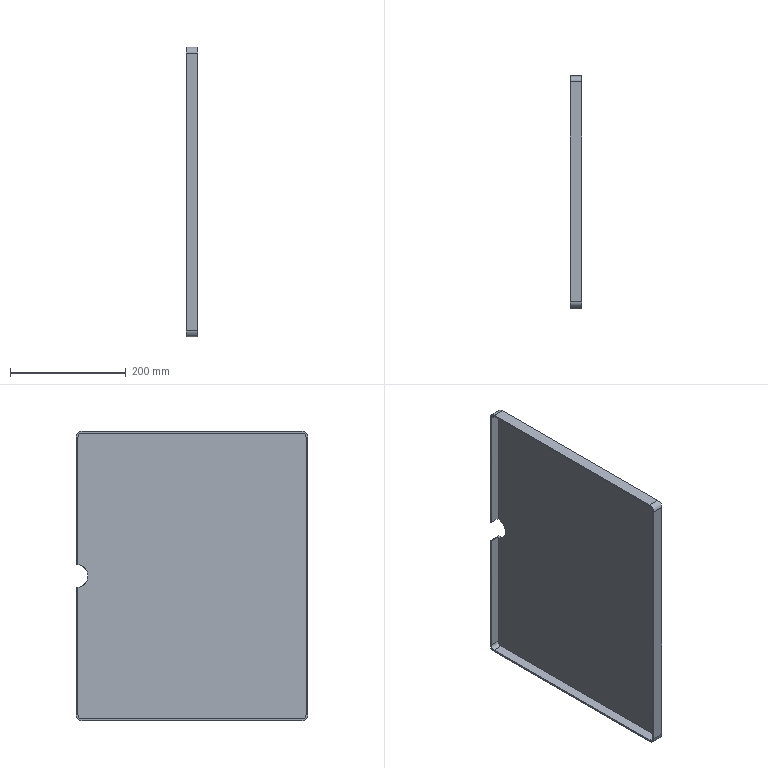Component | SolidWorks | LX-TSJ-17-1 | 1 solid | 22 faces | box 20 x 400 x 500 mm | volume 686219 mm3 | plane 13 | cylinder 9 | commonest cylinder face diameters 20 x4 14 x4 40.343 x1
STEP:
#1=COLOUR_RGB('',0.7922,0.8196,0.9333);
#2=FILL_AREA_STYLE_COLOUR('',#1);
#3=FILL_AREA_STYLE('',(#2));
#4=SURFACE_STYLE_FILL_AREA(#3);
#5=SURFACE_SIDE_STYLE('',(#4));
#6=SURFACE_STYLE_USAGE(.BOTH.,#5);
#7=PRESENTATION_STYLE_ASSIGNMENT((#6));
#8=CARTESIAN_POINT('',(4.999,-15.234,-15.481));
#9=VERTEX_POINT('',#8);
#10=CARTESIAN_POINT('',(4.999,-15.234,-17.069));
#11=VERTEX_POINT('',#10);
#12=CARTESIAN_POINT('',(4.999,-15.234,-16.275));
#13=DIRECTION('',(1.,0.,-0.));
#14=DIRECTION('',(-0.,0.,-1.));
#15=AXIS2_PLACEMENT_3D('',#12,#13,#14);
#16=CIRCLE('',#15,0.7941);
#17=EDGE_CURVE('',#9,#11,#16,.T.);
#18=ORIENTED_EDGE('',*,*,#17,.F.);
#19=CARTESIAN_POINT('',(4.999,-15.234,-6.826));
#20=VERTEX_POINT('',#19);
#21=CARTESIAN_POINT('',(4.999,-15.234,-25.724));
#22=DIRECTION('',(-0.,0.,-1.));
#23=VECTOR('',#22,39.37);
#24=LINE('',#21,#23);
#25=EDGE_CURVE('',#20,#9,#24,.T.);
#26=ORIENTED_EDGE('',*,*,#25,.F.);
#27=CARTESIAN_POINT('',(4.999,-15.627,-6.433));
#28=VERTEX_POINT('',#27);
#29=CARTESIAN_POINT('',(4.999,-15.627,-6.826));
#30=DIRECTION('',(-1.,0.,0.));
#31=DIRECTION('',(-0.,0.,-1.));
#32=AXIS2_PLACEMENT_3D('',#29,#30,#31);
#33=CIRCLE('',#32,0.3937);
#34=EDGE_CURVE('',#28,#20,#33,.T.);
#35=ORIENTED_EDGE('',*,*,#34,.F.);
#36=CARTESIAN_POINT('',(4.999,-30.588,-6.433));
#37=VERTEX_POINT('',#36);
#38=CARTESIAN_POINT('',(4.999,-30.588,-6.433));
#39=DIRECTION('',(0.,1.,0.));
#40=VECTOR('',#39,39.37);
#41=LINE('',#38,#40);
#42=EDGE_CURVE('',#37,#28,#41,.T.);
#43=ORIENTED_EDGE('',*,*,#42,.F.);
#44=CARTESIAN_POINT('',(4.999,-30.982,-6.826));
#45=VERTEX_POINT('',#44);
#46=CARTESIAN_POINT('',(4.999,-30.588,-6.826));
#47=DIRECTION('',(-1.,0.,0.));
#48=DIRECTION('',(-0.,0.,-1.));
#49=AXIS2_PLACEMENT_3D('',#46,#47,#48);
#50=CIRCLE('',#49,0.3937);
#51=EDGE_CURVE('',#45,#37,#50,.T.);
#52=ORIENTED_EDGE('',*,*,#51,.F.);
#53=CARTESIAN_POINT('',(4.999,-30.982,-25.724));
#54=VERTEX_POINT('',#53);
#55=CARTESIAN_POINT('',(4.999,-30.982,-25.724));
#56=DIRECTION('',(0.,0.,1.));
#57=VECTOR('',#56,39.37);
#58=LINE('',#55,#57);
#59=EDGE_CURVE('',#54,#45,#58,.T.);
#60=ORIENTED_EDGE('',*,*,#59,.F.);
#61=CARTESIAN_POINT('',(4.999,-30.588,-26.118));
#62=VERTEX_POINT('',#61);
#63=CARTESIAN_POINT('',(4.999,-30.588,-25.724));
#64=DIRECTION('',(-1.,0.,0.));
#65=DIRECTION('',(-0.,0.,-1.));
#66=AXIS2_PLACEMENT_3D('',#63,#64,#65);
#67=CIRCLE('',#66,0.3937);
#68=EDGE_CURVE('',#62,#54,#67,.T.);
#69=ORIENTED_EDGE('',*,*,#68,.F.);
#70=CARTESIAN_POINT('',(4.999,-15.627,-26.118));
#71=VERTEX_POINT('',#70);
#72=CARTESIAN_POINT('',(4.999,-30.588,-26.118));
#73=DIRECTION('',(0.,-1.,0.));
#74=VECTOR('',#73,39.37);
#75=LINE('',#72,#74);
#76=EDGE_CURVE('',#71,#62,#75,.T.);
#77=ORIENTED_EDGE('',*,*,#76,.F.);
#78=CARTESIAN_POINT('',(4.999,-15.234,-25.724));
#79=VERTEX_POINT('',#78);
#80=CARTESIAN_POINT('',(4.999,-15.627,-25.724));
#81=DIRECTION('',(-1.,0.,0.));
#82=DIRECTION('',(-0.,0.,-1.));
#83=AXIS2_PLACEMENT_3D('',#80,#81,#82);
#84=CIRCLE('',#83,0.3937);
#85=EDGE_CURVE('',#79,#71,#84,.T.);
#86=ORIENTED_EDGE('',*,*,#85,.F.);
#87=CARTESIAN_POINT('',(4.999,-15.234,-25.724));
#88=DIRECTION('',(-0.,0.,-1.));
#89=VECTOR('',#88,39.37);
#90=LINE('',#87,#89);
#91=EDGE_CURVE('',#11,#79,#90,.T.);
#92=ORIENTED_EDGE('',*,*,#91,.F.);
#93=EDGE_LOOP('',(#18,#26,#35,#43,#52,#60,#69,#77,#86,#92));
#94=FACE_OUTER_BOUND('',#93,.T.);
#95=CARTESIAN_POINT('',(4.999,-30.588,-25.724));
#96=DIRECTION('',(-1.,0.,0.));
#97=DIRECTION('',(0.,0.,1.));
#98=AXIS2_PLACEMENT_3D('',#95,#96,#97);
#99=PLANE('',#98);
#100=ADVANCED_FACE('',(#94),#99,.F.);
#101=CARTESIAN_POINT('',(4.212,-15.234,-17.069));
#102=VERTEX_POINT('',#101);
#103=CARTESIAN_POINT('',(4.212,-15.234,-17.069));
#104=DIRECTION('',(-1.,0.,0.));
#105=VECTOR('',#104,39.37);
#106=LINE('',#103,#105);
#107=EDGE_CURVE('',#11,#102,#106,.T.);
#108=ORIENTED_EDGE('',*,*,#107,.F.);
#109=ORIENTED_EDGE('',*,*,#91,.T.);
#110=CARTESIAN_POINT('',(4.212,-15.234,-25.724));
#111=VERTEX_POINT('',#110);
#112=CARTESIAN_POINT('',(4.212,-15.234,-25.724));
#113=DIRECTION('',(1.,0.,-0.));
#114=VECTOR('',#113,39.37);
#115=LINE('',#112,#114);
#116=EDGE_CURVE('',#111,#79,#115,.T.);
#117=ORIENTED_EDGE('',*,*,#116,.F.);
#118=CARTESIAN_POINT('',(4.212,-15.234,-25.724));
#119=DIRECTION('',(-0.,0.,-1.));
#120=VECTOR('',#119,39.37);
#121=LINE('',#118,#120);
#122=EDGE_CURVE('',#102,#111,#121,.T.);
#123=ORIENTED_EDGE('',*,*,#122,.F.);
#124=EDGE_LOOP('',(#108,#109,#117,#123));
#125=FACE_OUTER_BOUND('',#124,.T.);
#126=CARTESIAN_POINT('',(4.212,-15.234,-25.724));
#127=DIRECTION('',(0.,-1.,0.));
#128=DIRECTION('',(1.,0.,-0.));
#129=AXIS2_PLACEMENT_3D('',#126,#127,#128);
#130=PLANE('',#129);
#131=ADVANCED_FACE('',(#125),#130,.F.);
#132=CARTESIAN_POINT('',(4.881,-15.352,-17.061));
#133=VERTEX_POINT('',#132);
#134=CARTESIAN_POINT('',(4.212,-15.352,-17.061));
#135=VERTEX_POINT('',#134);
#136=CARTESIAN_POINT('',(4.212,-15.352,-17.061));
#137=DIRECTION('',(-1.,0.,0.));
#138=VECTOR('',#137,39.37);
#139=LINE('',#136,#138);
#140=EDGE_CURVE('',#133,#135,#139,.T.);
#141=ORIENTED_EDGE('',*,*,#140,.F.);
#142=CARTESIAN_POINT('',(4.881,-15.352,-15.49));
#143=VERTEX_POINT('',#142);
#144=CARTESIAN_POINT('',(4.881,-15.234,-16.275));
#145=DIRECTION('',(1.,0.,-0.));
#146=DIRECTION('',(-0.,0.,-1.));
#147=AXIS2_PLACEMENT_3D('',#144,#145,#146);
#148=CIRCLE('',#147,0.7941);
#149=EDGE_CURVE('',#143,#133,#148,.T.);
#150=ORIENTED_EDGE('',*,*,#149,.F.);
#151=CARTESIAN_POINT('',(4.212,-15.352,-15.49));
#152=VERTEX_POINT('',#151);
#153=CARTESIAN_POINT('',(4.212,-15.352,-15.49));
#154=DIRECTION('',(1.,0.,-0.));
#155=VECTOR('',#154,39.37);
#156=LINE('',#153,#155);
#157=EDGE_CURVE('',#152,#143,#156,.T.);
#158=ORIENTED_EDGE('',*,*,#157,.F.);
#159=CARTESIAN_POINT('',(4.212,-15.234,-15.481));
#160=VERTEX_POINT('',#159);
#161=CARTESIAN_POINT('',(4.212,-15.234,-16.275));
#162=DIRECTION('',(1.,0.,-0.));
#163=DIRECTION('',(-0.,0.,-1.));
#164=AXIS2_PLACEMENT_3D('',#161,#162,#163);
#165=CIRCLE('',#164,0.7941);
#166=EDGE_CURVE('',#160,#152,#165,.T.);
#167=ORIENTED_EDGE('',*,*,#166,.F.);
#168=CARTESIAN_POINT('',(4.212,-15.234,-15.481));
#169=DIRECTION('',(-1.,0.,0.));
#170=VECTOR('',#169,39.37);
#171=LINE('',#168,#170);
#172=EDGE_CURVE('',#9,#160,#171,.T.);
#173=ORIENTED_EDGE('',*,*,#172,.F.);
#174=ORIENTED_EDGE('',*,*,#17,.T.);
#175=ORIENTED_EDGE('',*,*,#107,.T.);
#176=CARTESIAN_POINT('',(4.212,-15.234,-16.275));
#177=DIRECTION('',(1.,0.,-0.));
#178=DIRECTION('',(-0.,0.,-1.));
#179=AXIS2_PLACEMENT_3D('',#176,#177,#178);
#180=CIRCLE('',#179,0.7941);
#181=EDGE_CURVE('',#135,#102,#180,.T.);
#182=ORIENTED_EDGE('',*,*,#181,.F.);
#183=EDGE_LOOP('',(#141,#150,#158,#167,#173,#174,#175,#182));
#184=FACE_OUTER_BOUND('',#183,.T.);
#185=CARTESIAN_POINT('',(4.212,-15.234,-16.275));
#186=DIRECTION('',(1.,0.,-0.));
#187=DIRECTION('',(-0.,0.,-1.));
#188=AXIS2_PLACEMENT_3D('',#185,#186,#187);
#189=CYLINDRICAL_SURFACE('',#188,0.7941);
#190=ADVANCED_FACE('',(#184),#189,.F.);
#191=ORIENTED_EDGE('',*,*,#172,.T.);
#192=CARTESIAN_POINT('',(4.212,-15.234,-6.826));
#193=VERTEX_POINT('',#192);
#194=CARTESIAN_POINT('',(4.212,-15.234,-25.724));
#195=DIRECTION('',(-0.,0.,-1.));
#196=VECTOR('',#195,39.37);
#197=LINE('',#194,#196);
#198=EDGE_CURVE('',#193,#160,#197,.T.);
#199=ORIENTED_EDGE('',*,*,#198,.F.);
#200=CARTESIAN_POINT('',(4.212,-15.234,-6.826));
#201=DIRECTION('',(-1.,0.,0.));
#202=VECTOR('',#201,39.37);
#203=LINE('',#200,#202);
#204=EDGE_CURVE('',#20,#193,#203,.T.);
#205=ORIENTED_EDGE('',*,*,#204,.F.);
#206=ORIENTED_EDGE('',*,*,#25,.T.);
#207=EDGE_LOOP('',(#191,#199,#205,#206));
#208=FACE_OUTER_BOUND('',#207,.T.);
#209=CARTESIAN_POINT('',(4.212,-15.234,-25.724));
#210=DIRECTION('',(0.,-1.,0.));
#211=DIRECTION('',(1.,0.,-0.));
#212=AXIS2_PLACEMENT_3D('',#209,#210,#211);
#213=PLANE('',#212);
#214=ADVANCED_FACE('',(#208),#213,.F.);
#215=CARTESIAN_POINT('',(4.212,-15.627,-6.433));
#216=VERTEX_POINT('',#215);
#217=CARTESIAN_POINT('',(4.212,-15.627,-6.826));
#218=DIRECTION('',(1.,0.,-0.));
#219=DIRECTION('',(-0.,0.,-1.));
#220=AXIS2_PLACEMENT_3D('',#217,#218,#219);
#221=CIRCLE('',#220,0.3937);
#222=EDGE_CURVE('',#193,#216,#221,.T.);
#223=ORIENTED_EDGE('',*,*,#222,.T.);
#224=CARTESIAN_POINT('',(4.212,-15.627,-6.433));
#225=DIRECTION('',(1.,0.,-0.));
#226=VECTOR('',#225,39.37);
#227=LINE('',#224,#226);
#228=EDGE_CURVE('',#216,#28,#227,.T.);
#229=ORIENTED_EDGE('',*,*,#228,.T.);
#230=ORIENTED_EDGE('',*,*,#34,.T.);
#231=ORIENTED_EDGE('',*,*,#204,.T.);
#232=EDGE_LOOP('',(#223,#229,#230,#231));
#233=FACE_OUTER_BOUND('',#232,.T.);
#234=CARTESIAN_POINT('',(4.212,-15.627,-6.826));
#235=DIRECTION('',(1.,0.,-0.));
#236=DIRECTION('',(-0.,0.,-1.));
#237=AXIS2_PLACEMENT_3D('',#234,#235,#236);
#238=CYLINDRICAL_SURFACE('',#237,0.3937);
#239=ADVANCED_FACE('',(#233),#238,.T.);
#240=ORIENTED_EDGE('',*,*,#228,.F.);
#241=CARTESIAN_POINT('',(4.212,-30.588,-6.433));
#242=VERTEX_POINT('',#241);
#243=CARTESIAN_POINT('',(4.212,-15.627,-6.433));
#244=DIRECTION('',(-0.,1.,-0.));
#245=VECTOR('',#244,39.37);
#246=LINE('',#243,#245);
#247=EDGE_CURVE('',#242,#216,#246,.T.);
#248=ORIENTED_EDGE('',*,*,#247,.F.);
#249=CARTESIAN_POINT('',(4.212,-30.588,-6.433));
#250=DIRECTION('',(-1.,0.,0.));
#251=VECTOR('',#250,39.37);
#252=LINE('',#249,#251);
#253=EDGE_CURVE('',#37,#242,#252,.T.);
#254=ORIENTED_EDGE('',*,*,#253,.F.);
#255=ORIENTED_EDGE('',*,*,#42,.T.);
#256=EDGE_LOOP('',(#240,#248,#254,#255));
#257=FACE_OUTER_BOUND('',#256,.T.);
#258=CARTESIAN_POINT('',(4.212,-15.627,-6.433));
#259=DIRECTION('',(-0.,-0.,-1.));
#260=DIRECTION('',(0.,-1.,0.));
#261=AXIS2_PLACEMENT_3D('',#258,#259,#260);
#262=PLANE('',#261);
#263=ADVANCED_FACE('',(#257),#262,.F.);
#264=CARTESIAN_POINT('',(4.212,-30.982,-6.826));
#265=VERTEX_POINT('',#264);
#266=CARTESIAN_POINT('',(4.212,-30.588,-6.826));
#267=DIRECTION('',(1.,0.,-0.));
#268=DIRECTION('',(-0.,0.,-1.));
#269=AXIS2_PLACEMENT_3D('',#266,#267,#268);
#270=CIRCLE('',#269,0.3937);
#271=EDGE_CURVE('',#242,#265,#270,.T.);
#272=ORIENTED_EDGE('',*,*,#271,.T.);
#273=CARTESIAN_POINT('',(4.212,-30.982,-6.826));
#274=DIRECTION('',(1.,0.,-0.));
#275=VECTOR('',#274,39.37);
#276=LINE('',#273,#275);
#277=EDGE_CURVE('',#265,#45,#276,.T.);
#278=ORIENTED_EDGE('',*,*,#277,.T.);
#279=ORIENTED_EDGE('',*,*,#51,.T.);
#280=ORIENTED_EDGE('',*,*,#253,.T.);
#281=EDGE_LOOP('',(#272,#278,#279,#280));
#282=FACE_OUTER_BOUND('',#281,.T.);
#283=CARTESIAN_POINT('',(4.212,-30.588,-6.826));
#284=DIRECTION('',(1.,0.,-0.));
#285=DIRECTION('',(-0.,0.,-1.));
#286=AXIS2_PLACEMENT_3D('',#283,#284,#285);
#287=CYLINDRICAL_SURFACE('',#286,0.3937);
#288=ADVANCED_FACE('',(#282),#287,.T.);
#289=ORIENTED_EDGE('',*,*,#277,.F.);
#290=CARTESIAN_POINT('',(4.212,-30.982,-25.724));
#291=VERTEX_POINT('',#290);
#292=CARTESIAN_POINT('',(4.212,-30.982,-25.724));
#293=DIRECTION('',(0.,0.,1.));
#294=VECTOR('',#293,39.37);
#295=LINE('',#292,#294);
#296=EDGE_CURVE('',#291,#265,#295,.T.);
#297=ORIENTED_EDGE('',*,*,#296,.F.);
#298=CARTESIAN_POINT('',(4.212,-30.982,-25.724));
#299=DIRECTION('',(-1.,0.,0.));
#300=VECTOR('',#299,39.37);
#301=LINE('',#298,#300);
#302=EDGE_CURVE('',#54,#291,#301,.T.);
#303=ORIENTED_EDGE('',*,*,#302,.F.);
#304=ORIENTED_EDGE('',*,*,#59,.T.);
#305=EDGE_LOOP('',(#289,#297,#303,#304));
#306=FACE_OUTER_BOUND('',#305,.T.);
#307=CARTESIAN_POINT('',(4.212,-30.982,-25.724));
#308=DIRECTION('',(0.,1.,0.));
#309=DIRECTION('',(-1.,0.,0.));
#310=AXIS2_PLACEMENT_3D('',#307,#308,#309);
#311=PLANE('',#310);
#312=ADVANCED_FACE('',(#306),#311,.F.);
#313=CARTESIAN_POINT('',(4.212,-30.588,-26.118));
#314=VERTEX_POINT('',#313);
#315=CARTESIAN_POINT('',(4.212,-30.588,-25.724));
#316=DIRECTION('',(1.,0.,-0.));
#317=DIRECTION('',(-0.,0.,-1.));
#318=AXIS2_PLACEMENT_3D('',#315,#316,#317);
#319=CIRCLE('',#318,0.3937);
#320=EDGE_CURVE('',#291,#314,#319,.T.);
#321=ORIENTED_EDGE('',*,*,#320,.T.);
#322=CARTESIAN_POINT('',(4.212,-30.588,-26.118));
#323=DIRECTION('',(1.,0.,-0.));
#324=VECTOR('',#323,39.37);
#325=LINE('',#322,#324);
#326=EDGE_CURVE('',#314,#62,#325,.T.);
#327=ORIENTED_EDGE('',*,*,#326,.T.);
#328=ORIENTED_EDGE('',*,*,#68,.T.);
#329=ORIENTED_EDGE('',*,*,#302,.T.);
#330=EDGE_LOOP('',(#321,#327,#328,#329));
#331=FACE_OUTER_BOUND('',#330,.T.);
#332=CARTESIAN_POINT('',(4.212,-30.588,-25.724));
#333=DIRECTION('',(1.,0.,-0.));
#334=DIRECTION('',(-0.,0.,-1.));
#335=AXIS2_PLACEMENT_3D('',#332,#333,#334);
#336=CYLINDRICAL_SURFACE('',#335,0.3937);
#337=ADVANCED_FACE('',(#331),#336,.T.);
#338=ORIENTED_EDGE('',*,*,#326,.F.);
#339=CARTESIAN_POINT('',(4.212,-15.627,-26.118));
#340=VERTEX_POINT('',#339);
#341=CARTESIAN_POINT('',(4.212,-15.627,-26.118));
#342=DIRECTION('',(0.,-1.,0.));
#343=VECTOR('',#342,39.37);
#344=LINE('',#341,#343);
#345=EDGE_CURVE('',#340,#314,#344,.T.);
#346=ORIENTED_EDGE('',*,*,#345,.F.);
#347=CARTESIAN_POINT('',(4.212,-15.627,-26.118));
#348=DIRECTION('',(-1.,0.,0.));
#349=VECTOR('',#348,39.37);
#350=LINE('',#347,#349);
#351=EDGE_CURVE('',#71,#340,#350,.T.);
#352=ORIENTED_EDGE('',*,*,#351,.F.);
#353=ORIENTED_EDGE('',*,*,#76,.T.);
#354=EDGE_LOOP('',(#338,#346,#352,#353));
#355=FACE_OUTER_BOUND('',#354,.T.);
#356=CARTESIAN_POINT('',(4.212,-15.627,-26.118));
#357=DIRECTION('',(0.,0.,1.));
#358=DIRECTION('',(-0.,1.,-0.));
#359=AXIS2_PLACEMENT_3D('',#356,#357,#358);
#360=PLANE('',#359);
#361=ADVANCED_FACE('',(#355),#360,.F.);
#362=CARTESIAN_POINT('',(4.212,-15.627,-25.724));
#363=DIRECTION('',(1.,0.,-0.));
#364=DIRECTION('',(-0.,0.,-1.));
#365=AXIS2_PLACEMENT_3D('',#362,#363,#364);
#366=CIRCLE('',#365,0.3937);
#367=EDGE_CURVE('',#340,#111,#366,.T.);
#368=ORIENTED_EDGE('',*,*,#367,.T.);
#369=ORIENTED_EDGE('',*,*,#116,.T.);
#370=ORIENTED_EDGE('',*,*,#85,.T.);
#371=ORIENTED_EDGE('',*,*,#351,.T.);
#372=EDGE_LOOP('',(#368,#369,#370,#371));
#373=FACE_OUTER_BOUND('',#372,.T.);
#374=CARTESIAN_POINT('',(4.212,-15.627,-25.724));
#375=DIRECTION('',(1.,0.,-0.));
#376=DIRECTION('',(-0.,0.,-1.));
#377=AXIS2_PLACEMENT_3D('',#374,#375,#376);
#378=CYLINDRICAL_SURFACE('',#377,0.3937);
#379=ADVANCED_FACE('',(#373),#378,.T.);
#380=CARTESIAN_POINT('',(4.212,-15.627,-26.));
#381=VERTEX_POINT('',#380);
#382=CARTESIAN_POINT('',(4.212,-15.352,-25.724));
#383=VERTEX_POINT('',#382);
#384=CARTESIAN_POINT('',(4.212,-15.627,-25.724));
#385=DIRECTION('',(1.,0.,-0.));
#386=DIRECTION('',(-0.,0.,-1.));
#387=AXIS2_PLACEMENT_3D('',#384,#385,#386);
#388=CIRCLE('',#387,0.2756);
#389=EDGE_CURVE('',#381,#383,#388,.T.);
#390=ORIENTED_EDGE('',*,*,#389,.T.);
#391=CARTESIAN_POINT('',(4.212,-15.352,-25.724));
#392=DIRECTION('',(0.,0.,1.));
#393=VECTOR('',#392,39.37);
#394=LINE('',#391,#393);
#395=EDGE_CURVE('',#383,#135,#394,.T.);
#396=ORIENTED_EDGE('',*,*,#395,.T.);
#397=ORIENTED_EDGE('',*,*,#181,.T.);
#398=ORIENTED_EDGE('',*,*,#122,.T.);
#399=ORIENTED_EDGE('',*,*,#367,.F.);
#400=ORIENTED_EDGE('',*,*,#345,.T.);
#401=ORIENTED_EDGE('',*,*,#320,.F.);
#402=ORIENTED_EDGE('',*,*,#296,.T.);
#403=ORIENTED_EDGE('',*,*,#271,.F.);
#404=ORIENTED_EDGE('',*,*,#247,.T.);
#405=ORIENTED_EDGE('',*,*,#222,.F.);
#406=ORIENTED_EDGE('',*,*,#198,.T.);
#407=ORIENTED_EDGE('',*,*,#166,.T.);
#408=CARTESIAN_POINT('',(4.212,-15.352,-6.826));
#409=VERTEX_POINT('',#408);
#410=CARTESIAN_POINT('',(4.212,-15.352,-25.724));
#411=DIRECTION('',(0.,0.,1.));
#412=VECTOR('',#411,39.37);
#413=LINE('',#410,#412);
#414=EDGE_CURVE('',#152,#409,#413,.T.);
#415=ORIENTED_EDGE('',*,*,#414,.T.);
#416=CARTESIAN_POINT('',(4.212,-15.627,-6.551));
#417=VERTEX_POINT('',#416);
#418=CARTESIAN_POINT('',(4.212,-15.627,-6.826));
#419=DIRECTION('',(1.,0.,-0.));
#420=DIRECTION('',(-0.,0.,-1.));
#421=AXIS2_PLACEMENT_3D('',#418,#419,#420);
#422=CIRCLE('',#421,0.2756);
#423=EDGE_CURVE('',#409,#417,#422,.T.);
#424=ORIENTED_EDGE('',*,*,#423,.T.);
#425=CARTESIAN_POINT('',(4.212,-30.588,-6.551));
#426=VERTEX_POINT('',#425);
#427=CARTESIAN_POINT('',(4.212,-30.588,-6.551));
#428=DIRECTION('',(0.,-1.,0.));
#429=VECTOR('',#428,39.37);
#430=LINE('',#427,#429);
#431=EDGE_CURVE('',#417,#426,#430,.T.);
#432=ORIENTED_EDGE('',*,*,#431,.T.);
#433=CARTESIAN_POINT('',(4.212,-30.864,-6.826));
#434=VERTEX_POINT('',#433);
#435=CARTESIAN_POINT('',(4.212,-30.588,-6.826));
#436=DIRECTION('',(1.,0.,-0.));
#437=DIRECTION('',(-0.,0.,-1.));
#438=AXIS2_PLACEMENT_3D('',#435,#436,#437);
#439=CIRCLE('',#438,0.2756);
#440=EDGE_CURVE('',#426,#434,#439,.T.);
#441=ORIENTED_EDGE('',*,*,#440,.T.);
#442=CARTESIAN_POINT('',(4.212,-30.864,-25.724));
#443=VERTEX_POINT('',#442);
#444=CARTESIAN_POINT('',(4.212,-30.864,-25.724));
#445=DIRECTION('',(-0.,0.,-1.));
#446=VECTOR('',#445,39.37);
#447=LINE('',#444,#446);
#448=EDGE_CURVE('',#434,#443,#447,.T.);
#449=ORIENTED_EDGE('',*,*,#448,.T.);
#450=CARTESIAN_POINT('',(4.212,-30.588,-26.));
#451=VERTEX_POINT('',#450);
#452=CARTESIAN_POINT('',(4.212,-30.588,-25.724));
#453=DIRECTION('',(1.,0.,-0.));
#454=DIRECTION('',(-0.,0.,-1.));
#455=AXIS2_PLACEMENT_3D('',#452,#453,#454);
#456=CIRCLE('',#455,0.2756);
#457=EDGE_CURVE('',#443,#451,#456,.T.);
#458=ORIENTED_EDGE('',*,*,#457,.T.);
#459=CARTESIAN_POINT('',(4.212,-30.588,-26.));
#460=DIRECTION('',(0.,1.,0.));
#461=VECTOR('',#460,39.37);
#462=LINE('',#459,#461);
#463=EDGE_CURVE('',#451,#381,#462,.T.);
#464=ORIENTED_EDGE('',*,*,#463,.T.);
#465=EDGE_LOOP('',(#390,#396,#397,#398,#399,#400,#401,#402,#403,#404,#405,#406,#407,#415,#424,#432,#441,#449,#458,#464));
#466=FACE_OUTER_BOUND('',#465,.T.);
#467=CARTESIAN_POINT('',(4.212,-30.588,-25.724));
#468=DIRECTION('',(-1.,0.,0.));
#469=DIRECTION('',(0.,0.,1.));
#470=AXIS2_PLACEMENT_3D('',#467,#468,#469);
#471=PLANE('',#470);
#472=ADVANCED_FACE('',(#466),#471,.T.);
#473=CARTESIAN_POINT('',(4.881,-15.352,-25.724));
#474=VERTEX_POINT('',#473);
#475=CARTESIAN_POINT('',(4.212,-15.352,-25.724));
#476=DIRECTION('',(1.,0.,-0.));
#477=VECTOR('',#476,39.37);
#478=LINE('',#475,#477);
#479=EDGE_CURVE('',#383,#474,#478,.T.);
#480=ORIENTED_EDGE('',*,*,#479,.T.);
#481=CARTESIAN_POINT('',(4.881,-15.352,-25.724));
#482=DIRECTION('',(0.,0.,1.));
#483=VECTOR('',#482,39.37);
#484=LINE('',#481,#483);
#485=EDGE_CURVE('',#474,#133,#484,.T.);
#486=ORIENTED_EDGE('',*,*,#485,.T.);
#487=ORIENTED_EDGE('',*,*,#140,.T.);
#488=ORIENTED_EDGE('',*,*,#395,.F.);
#489=EDGE_LOOP('',(#480,#486,#487,#488));
#490=FACE_OUTER_BOUND('',#489,.T.);
#491=CARTESIAN_POINT('',(4.212,-15.352,-25.724));
#492=DIRECTION('',(0.,-1.,0.));
#493=DIRECTION('',(1.,0.,-0.));
#494=AXIS2_PLACEMENT_3D('',#491,#492,#493);
#495=PLANE('',#494);
#496=ADVANCED_FACE('',(#490),#495,.T.);
#497=CARTESIAN_POINT('',(4.881,-15.627,-6.551));
#498=VERTEX_POINT('',#497);
#499=CARTESIAN_POINT('',(4.881,-15.352,-6.826));
#500=VERTEX_POINT('',#499);
#501=CARTESIAN_POINT('',(4.881,-15.627,-6.826));
#502=DIRECTION('',(-1.,0.,0.));
#503=DIRECTION('',(-0.,0.,-1.));
#504=AXIS2_PLACEMENT_3D('',#501,#502,#503);
#505=CIRCLE('',#504,0.2756);
#506=EDGE_CURVE('',#498,#500,#505,.T.);
#507=ORIENTED_EDGE('',*,*,#506,.T.);
#508=CARTESIAN_POINT('',(4.881,-15.352,-25.724));
#509=DIRECTION('',(-0.,0.,-1.));
#510=VECTOR('',#509,39.37);
#511=LINE('',#508,#510);
#512=EDGE_CURVE('',#500,#143,#511,.T.);
#513=ORIENTED_EDGE('',*,*,#512,.T.);
#514=ORIENTED_EDGE('',*,*,#149,.T.);
#515=ORIENTED_EDGE('',*,*,#485,.F.);
#516=CARTESIAN_POINT('',(4.881,-15.627,-26.));
#517=VERTEX_POINT('',#516);
#518=CARTESIAN_POINT('',(4.881,-15.627,-25.724));
#519=DIRECTION('',(-1.,0.,0.));
#520=DIRECTION('',(-0.,0.,-1.));
#521=AXIS2_PLACEMENT_3D('',#518,#519,#520);
#522=CIRCLE('',#521,0.2756);
#523=EDGE_CURVE('',#474,#517,#522,.T.);
#524=ORIENTED_EDGE('',*,*,#523,.T.);
#525=CARTESIAN_POINT('',(4.881,-30.588,-26.));
#526=VERTEX_POINT('',#525);
#527=CARTESIAN_POINT('',(4.881,-30.588,-26.));
#528=DIRECTION('',(0.,-1.,0.));
#529=VECTOR('',#528,39.37);
#530=LINE('',#527,#529);
#531=EDGE_CURVE('',#517,#526,#530,.T.);
#532=ORIENTED_EDGE('',*,*,#531,.T.);
#533=CARTESIAN_POINT('',(4.881,-30.864,-25.724));
#534=VERTEX_POINT('',#533);
#535=CARTESIAN_POINT('',(4.881,-30.588,-25.724));
#536=DIRECTION('',(-1.,0.,0.));
#537=DIRECTION('',(-0.,0.,-1.));
#538=AXIS2_PLACEMENT_3D('',#535,#536,#537);
#539=CIRCLE('',#538,0.2756);
#540=EDGE_CURVE('',#526,#534,#539,.T.);
#541=ORIENTED_EDGE('',*,*,#540,.T.);
#542=CARTESIAN_POINT('',(4.881,-30.864,-6.826));
#543=VERTEX_POINT('',#542);
#544=CARTESIAN_POINT('',(4.881,-30.864,-25.724));
#545=DIRECTION('',(0.,0.,1.));
#546=VECTOR('',#545,39.37);
#547=LINE('',#544,#546);
#548=EDGE_CURVE('',#534,#543,#547,.T.);
#549=ORIENTED_EDGE('',*,*,#548,.T.);
#550=CARTESIAN_POINT('',(4.881,-30.588,-6.551));
#551=VERTEX_POINT('',#550);
#552=CARTESIAN_POINT('',(4.881,-30.588,-6.826));
#553=DIRECTION('',(-1.,0.,0.));
#554=DIRECTION('',(-0.,0.,-1.));
#555=AXIS2_PLACEMENT_3D('',#552,#553,#554);
#556=CIRCLE('',#555,0.2756);
#557=EDGE_CURVE('',#543,#551,#556,.T.);
#558=ORIENTED_EDGE('',*,*,#557,.T.);
#559=CARTESIAN_POINT('',(4.881,-30.588,-6.551));
#560=DIRECTION('',(0.,1.,0.));
#561=VECTOR('',#560,39.37);
#562=LINE('',#559,#561);
#563=EDGE_CURVE('',#551,#498,#562,.T.);
#564=ORIENTED_EDGE('',*,*,#563,.T.);
#565=EDGE_LOOP('',(#507,#513,#514,#515,#524,#532,#541,#549,#558,#564));
#566=FACE_OUTER_BOUND('',#565,.T.);
#567=CARTESIAN_POINT('',(4.881,-30.588,-25.724));
#568=DIRECTION('',(-1.,0.,0.));
#569=DIRECTION('',(0.,0.,1.));
#570=AXIS2_PLACEMENT_3D('',#567,#568,#569);
#571=PLANE('',#570);
#572=ADVANCED_FACE('',(#566),#571,.T.);
#573=CARTESIAN_POINT('',(4.212,-15.352,-6.826));
#574=DIRECTION('',(-1.,0.,0.));
#575=VECTOR('',#574,39.37);
#576=LINE('',#573,#575);
#577=EDGE_CURVE('',#500,#409,#576,.T.);
#578=ORIENTED_EDGE('',*,*,#577,.T.);
#579=ORIENTED_EDGE('',*,*,#414,.F.);
#580=ORIENTED_EDGE('',*,*,#157,.T.);
#581=ORIENTED_EDGE('',*,*,#512,.F.);
#582=EDGE_LOOP('',(#578,#579,#580,#581));
#583=FACE_OUTER_BOUND('',#582,.T.);
#584=CARTESIAN_POINT('',(4.212,-15.352,-25.724));
#585=DIRECTION('',(0.,-1.,0.));
#586=DIRECTION('',(1.,0.,-0.));
#587=AXIS2_PLACEMENT_3D('',#584,#585,#586);
#588=PLANE('',#587);
#589=ADVANCED_FACE('',(#583),#588,.T.);
#590=ORIENTED_EDGE('',*,*,#479,.F.);
#591=ORIENTED_EDGE('',*,*,#389,.F.);
#592=CARTESIAN_POINT('',(4.212,-15.627,-26.));
#593=DIRECTION('',(-1.,0.,0.));
#594=VECTOR('',#593,39.37);
#595=LINE('',#592,#594);
#596=EDGE_CURVE('',#517,#381,#595,.T.);
#597=ORIENTED_EDGE('',*,*,#596,.F.);
#598=ORIENTED_EDGE('',*,*,#523,.F.);
#599=EDGE_LOOP('',(#590,#591,#597,#598));
#600=FACE_OUTER_BOUND('',#599,.T.);
#601=CARTESIAN_POINT('',(4.212,-15.627,-25.724));
#602=DIRECTION('',(1.,0.,-0.));
#603=DIRECTION('',(-0.,0.,-1.));
#604=AXIS2_PLACEMENT_3D('',#601,#602,#603);
#605=CYLINDRICAL_SURFACE('',#604,0.2756);
#606=ADVANCED_FACE('',(#600),#605,.F.);
#607=ORIENTED_EDGE('',*,*,#463,.F.);
#608=CARTESIAN_POINT('',(4.212,-30.588,-26.));
#609=DIRECTION('',(1.,0.,-0.));
#610=VECTOR('',#609,39.37);
#611=LINE('',#608,#610);
#612=EDGE_CURVE('',#451,#526,#611,.T.);
#613=ORIENTED_EDGE('',*,*,#612,.T.);
#614=ORIENTED_EDGE('',*,*,#531,.F.);
#615=ORIENTED_EDGE('',*,*,#596,.T.);
#616=EDGE_LOOP('',(#607,#613,#614,#615));
#617=FACE_OUTER_BOUND('',#616,.T.);
#618=CARTESIAN_POINT('',(4.212,-15.627,-26.));
#619=DIRECTION('',(0.,0.,1.));
#620=DIRECTION('',(-0.,1.,-0.));
#621=AXIS2_PLACEMENT_3D('',#618,#619,#620);
#622=PLANE('',#621);
#623=ADVANCED_FACE('',(#617),#622,.T.);
#624=ORIENTED_EDGE('',*,*,#612,.F.);
#625=ORIENTED_EDGE('',*,*,#457,.F.);
#626=CARTESIAN_POINT('',(4.212,-30.864,-25.724));
#627=DIRECTION('',(-1.,0.,0.));
#628=VECTOR('',#627,39.37);
#629=LINE('',#626,#628);
#630=EDGE_CURVE('',#534,#443,#629,.T.);
#631=ORIENTED_EDGE('',*,*,#630,.F.);
#632=ORIENTED_EDGE('',*,*,#540,.F.);
#633=EDGE_LOOP('',(#624,#625,#631,#632));
#634=FACE_OUTER_BOUND('',#633,.T.);
#635=CARTESIAN_POINT('',(4.212,-30.588,-25.724));
#636=DIRECTION('',(1.,0.,-0.));
#637=DIRECTION('',(-0.,0.,-1.));
#638=AXIS2_PLACEMENT_3D('',#635,#636,#637);
#639=CYLINDRICAL_SURFACE('',#638,0.2756);
#640=ADVANCED_FACE('',(#634),#639,.F.);
#641=ORIENTED_EDGE('',*,*,#448,.F.);
#642=CARTESIAN_POINT('',(4.212,-30.864,-6.826));
#643=DIRECTION('',(1.,0.,-0.));
#644=VECTOR('',#643,39.37);
#645=LINE('',#642,#644);
#646=EDGE_CURVE('',#434,#543,#645,.T.);
#647=ORIENTED_EDGE('',*,*,#646,.T.);
#648=ORIENTED_EDGE('',*,*,#548,.F.);
#649=ORIENTED_EDGE('',*,*,#630,.T.);
#650=EDGE_LOOP('',(#641,#647,#648,#649));
#651=FACE_OUTER_BOUND('',#650,.T.);
#652=CARTESIAN_POINT('',(4.212,-30.864,-25.724));
#653=DIRECTION('',(0.,1.,0.));
#654=DIRECTION('',(-1.,0.,0.));
#655=AXIS2_PLACEMENT_3D('',#652,#653,#654);
#656=PLANE('',#655);
#657=ADVANCED_FACE('',(#651),#656,.T.);
#658=ORIENTED_EDGE('',*,*,#646,.F.);
#659=ORIENTED_EDGE('',*,*,#440,.F.);
#660=CARTESIAN_POINT('',(4.212,-30.588,-6.551));
#661=DIRECTION('',(-1.,0.,0.));
#662=VECTOR('',#661,39.37);
#663=LINE('',#660,#662);
#664=EDGE_CURVE('',#551,#426,#663,.T.);
#665=ORIENTED_EDGE('',*,*,#664,.F.);
#666=ORIENTED_EDGE('',*,*,#557,.F.);
#667=EDGE_LOOP('',(#658,#659,#665,#666));
#668=FACE_OUTER_BOUND('',#667,.T.);
#669=CARTESIAN_POINT('',(4.212,-30.588,-6.826));
#670=DIRECTION('',(1.,0.,-0.));
#671=DIRECTION('',(-0.,0.,-1.));
#672=AXIS2_PLACEMENT_3D('',#669,#670,#671);
#673=CYLINDRICAL_SURFACE('',#672,0.2756);
#674=ADVANCED_FACE('',(#668),#673,.F.);
#675=ORIENTED_EDGE('',*,*,#431,.F.);
#676=CARTESIAN_POINT('',(4.212,-15.627,-6.551));
#677=DIRECTION('',(1.,0.,-0.));
#678=VECTOR('',#677,39.37);
#679=LINE('',#676,#678);
#680=EDGE_CURVE('',#417,#498,#679,.T.);
#681=ORIENTED_EDGE('',*,*,#680,.T.);
#682=ORIENTED_EDGE('',*,*,#563,.F.);
#683=ORIENTED_EDGE('',*,*,#664,.T.);
#684=EDGE_LOOP('',(#675,#681,#682,#683));
#685=FACE_OUTER_BOUND('',#684,.T.);
#686=CARTESIAN_POINT('',(4.212,-15.627,-6.551));
#687=DIRECTION('',(-0.,-0.,-1.));
#688=DIRECTION('',(0.,-1.,0.));
#689=AXIS2_PLACEMENT_3D('',#686,#687,#688);
#690=PLANE('',#689);
#691=ADVANCED_FACE('',(#685),#690,.T.);
#692=ORIENTED_EDGE('',*,*,#680,.F.);
#693=ORIENTED_EDGE('',*,*,#423,.F.);
#694=ORIENTED_EDGE('',*,*,#577,.F.);
#695=ORIENTED_EDGE('',*,*,#506,.F.);
#696=EDGE_LOOP('',(#692,#693,#694,#695));
#697=FACE_OUTER_BOUND('',#696,.T.);
#698=CARTESIAN_POINT('',(4.212,-15.627,-6.826));
#699=DIRECTION('',(1.,0.,-0.));
#700=DIRECTION('',(-0.,0.,-1.));
#701=AXIS2_PLACEMENT_3D('',#698,#699,#700);
#702=CYLINDRICAL_SURFACE('',#701,0.2756);
#703=ADVANCED_FACE('',(#697),#702,.F.);
#704=CLOSED_SHELL('',(#100,#131,#190,#214,#239,#263,#288,#312,#337,#361,#379,#472,#496,#572,#589,#606,#623,#640,#657,#674,#691,#703));
#705=MANIFOLD_SOLID_BREP('',#704);
#706=STYLED_ITEM('',(#7),#705);
#707=PRESENTATION_LAYER_ASSIGNMENT('','',(#706));
#708=(LENGTH_UNIT()NAMED_UNIT(*)SI_UNIT($,.METRE.));
#709=LENGTH_MEASURE_WITH_UNIT(LENGTH_MEASURE(0.0254),#708);
#710=DIMENSIONAL_EXPONENTS(1.,0.,0.,0.,0.,0.,0.);
#711=(CONVERSION_BASED_UNIT('',#709)LENGTH_UNIT()NAMED_UNIT(#710));
#712=UNCERTAINTY_MEASURE_WITH_UNIT(LENGTH_MEASURE(0.00001),#711,'','');
#713=(NAMED_UNIT(*)PLANE_ANGLE_UNIT()SI_UNIT($,.RADIAN.));
#714=(NAMED_UNIT(*)SI_UNIT($,.STERADIAN.)SOLID_ANGLE_UNIT());
#715=(GEOMETRIC_REPRESENTATION_CONTEXT(3)GLOBAL_UNCERTAINTY_ASSIGNED_CONTEXT((#712))GLOBAL_UNIT_ASSIGNED_CONTEXT((#711,#713,#714))REPRESENTATION_CONTEXT('',''));
#716=MECHANICAL_DESIGN_GEOMETRIC_PRESENTATION_REPRESENTATION('',(#706),#715);
#717=CARTESIAN_POINT('',(0.,0.,0.));
#718=DIRECTION('',(0.,0.,1.));
#719=DIRECTION('',(1.,0.,0.));
#720=AXIS2_PLACEMENT_3D('',#717,#718,#719);
#721=(LENGTH_UNIT()NAMED_UNIT(*)SI_UNIT($,.METRE.));
#722=LENGTH_MEASURE_WITH_UNIT(LENGTH_MEASURE(0.0254),#721);
#723=DIMENSIONAL_EXPONENTS(1.,0.,0.,0.,0.,0.,0.);
#724=(CONVERSION_BASED_UNIT('',#722)LENGTH_UNIT()NAMED_UNIT(#723));
#725=UNCERTAINTY_MEASURE_WITH_UNIT(LENGTH_MEASURE(0.00001),#724,'','');
#726=(NAMED_UNIT(*)PLANE_ANGLE_UNIT()SI_UNIT($,.RADIAN.));
#727=(NAMED_UNIT(*)SI_UNIT($,.STERADIAN.)SOLID_ANGLE_UNIT());
#728=(GEOMETRIC_REPRESENTATION_CONTEXT(3)GLOBAL_UNCERTAINTY_ASSIGNED_CONTEXT((#725))GLOBAL_UNIT_ASSIGNED_CONTEXT((#724,#726,#727))REPRESENTATION_CONTEXT('',''));
#729=ADVANCED_BREP_SHAPE_REPRESENTATION('',(#705,#720),#728);